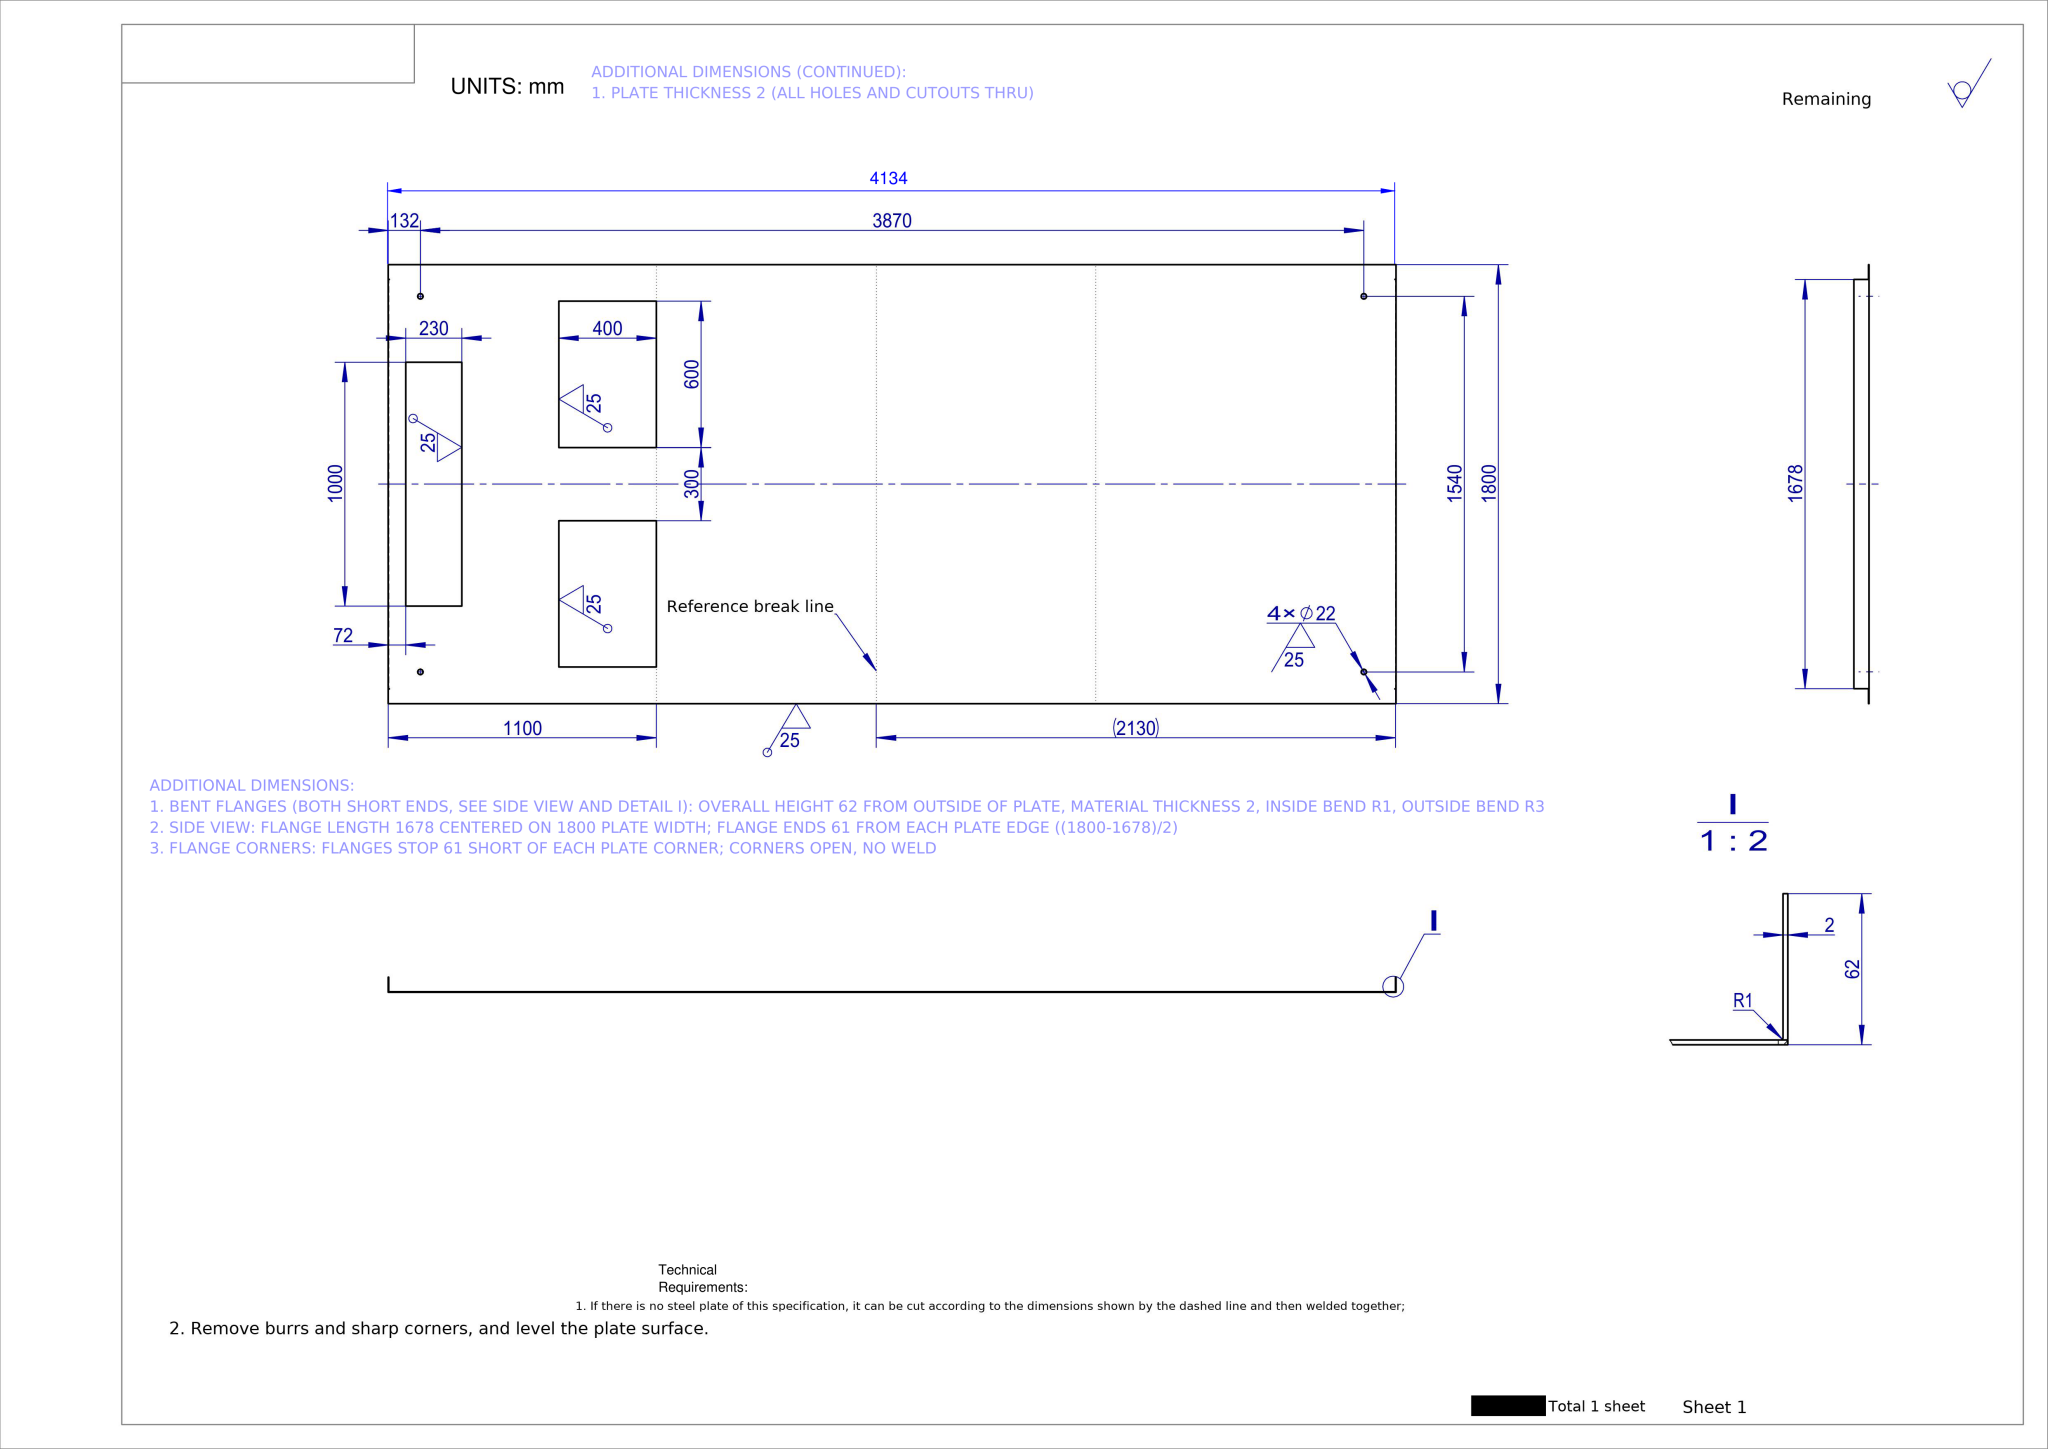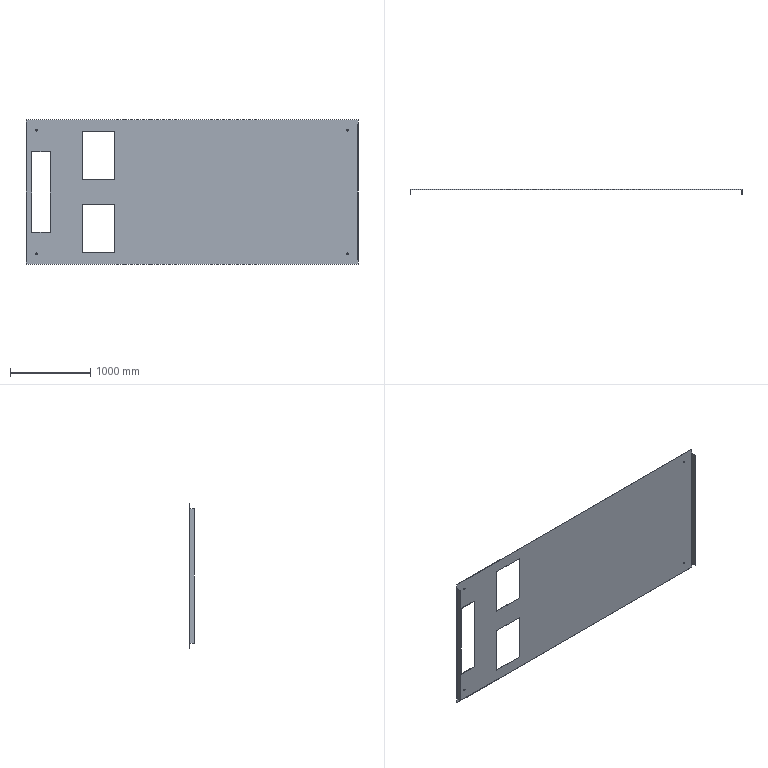Part | NX | mm | 1 solid | 58 faces | box 4134 x 62 x 1800 mm | volume 13856285 mm3 | plane 46 | cylinder 12 | commonest cylinder face diameters 22 x8 6 x2 2 x2